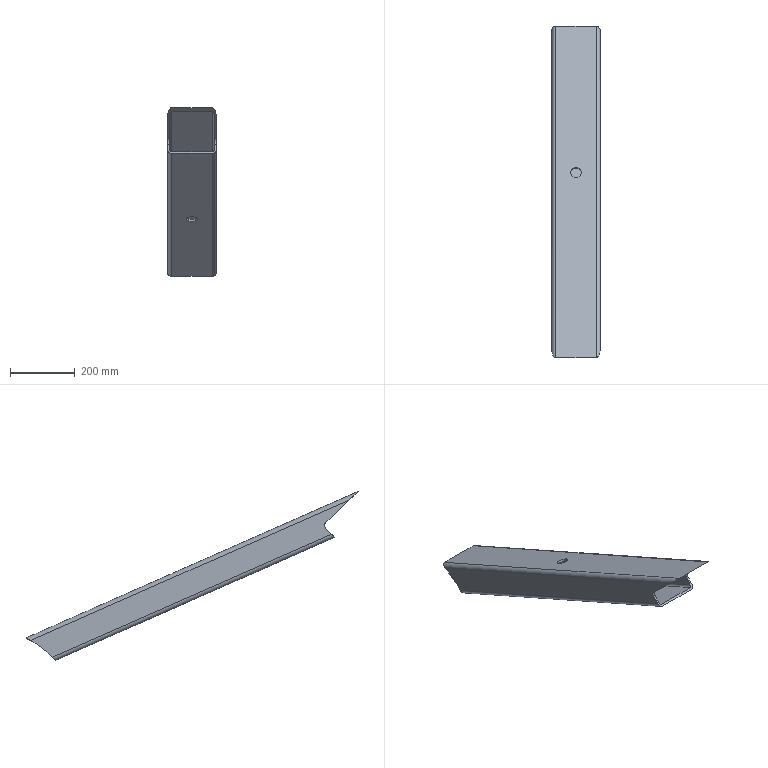Component | SolidWorks | Spona-7 | 1 solid | 25 faces | volume 2911339 mm3 | cylinder 15 | plane 10 | commonest cylinder face diameters 25.2 x6 34 x4 12.6 x4 601 x1 | material Plain Carbon Steel